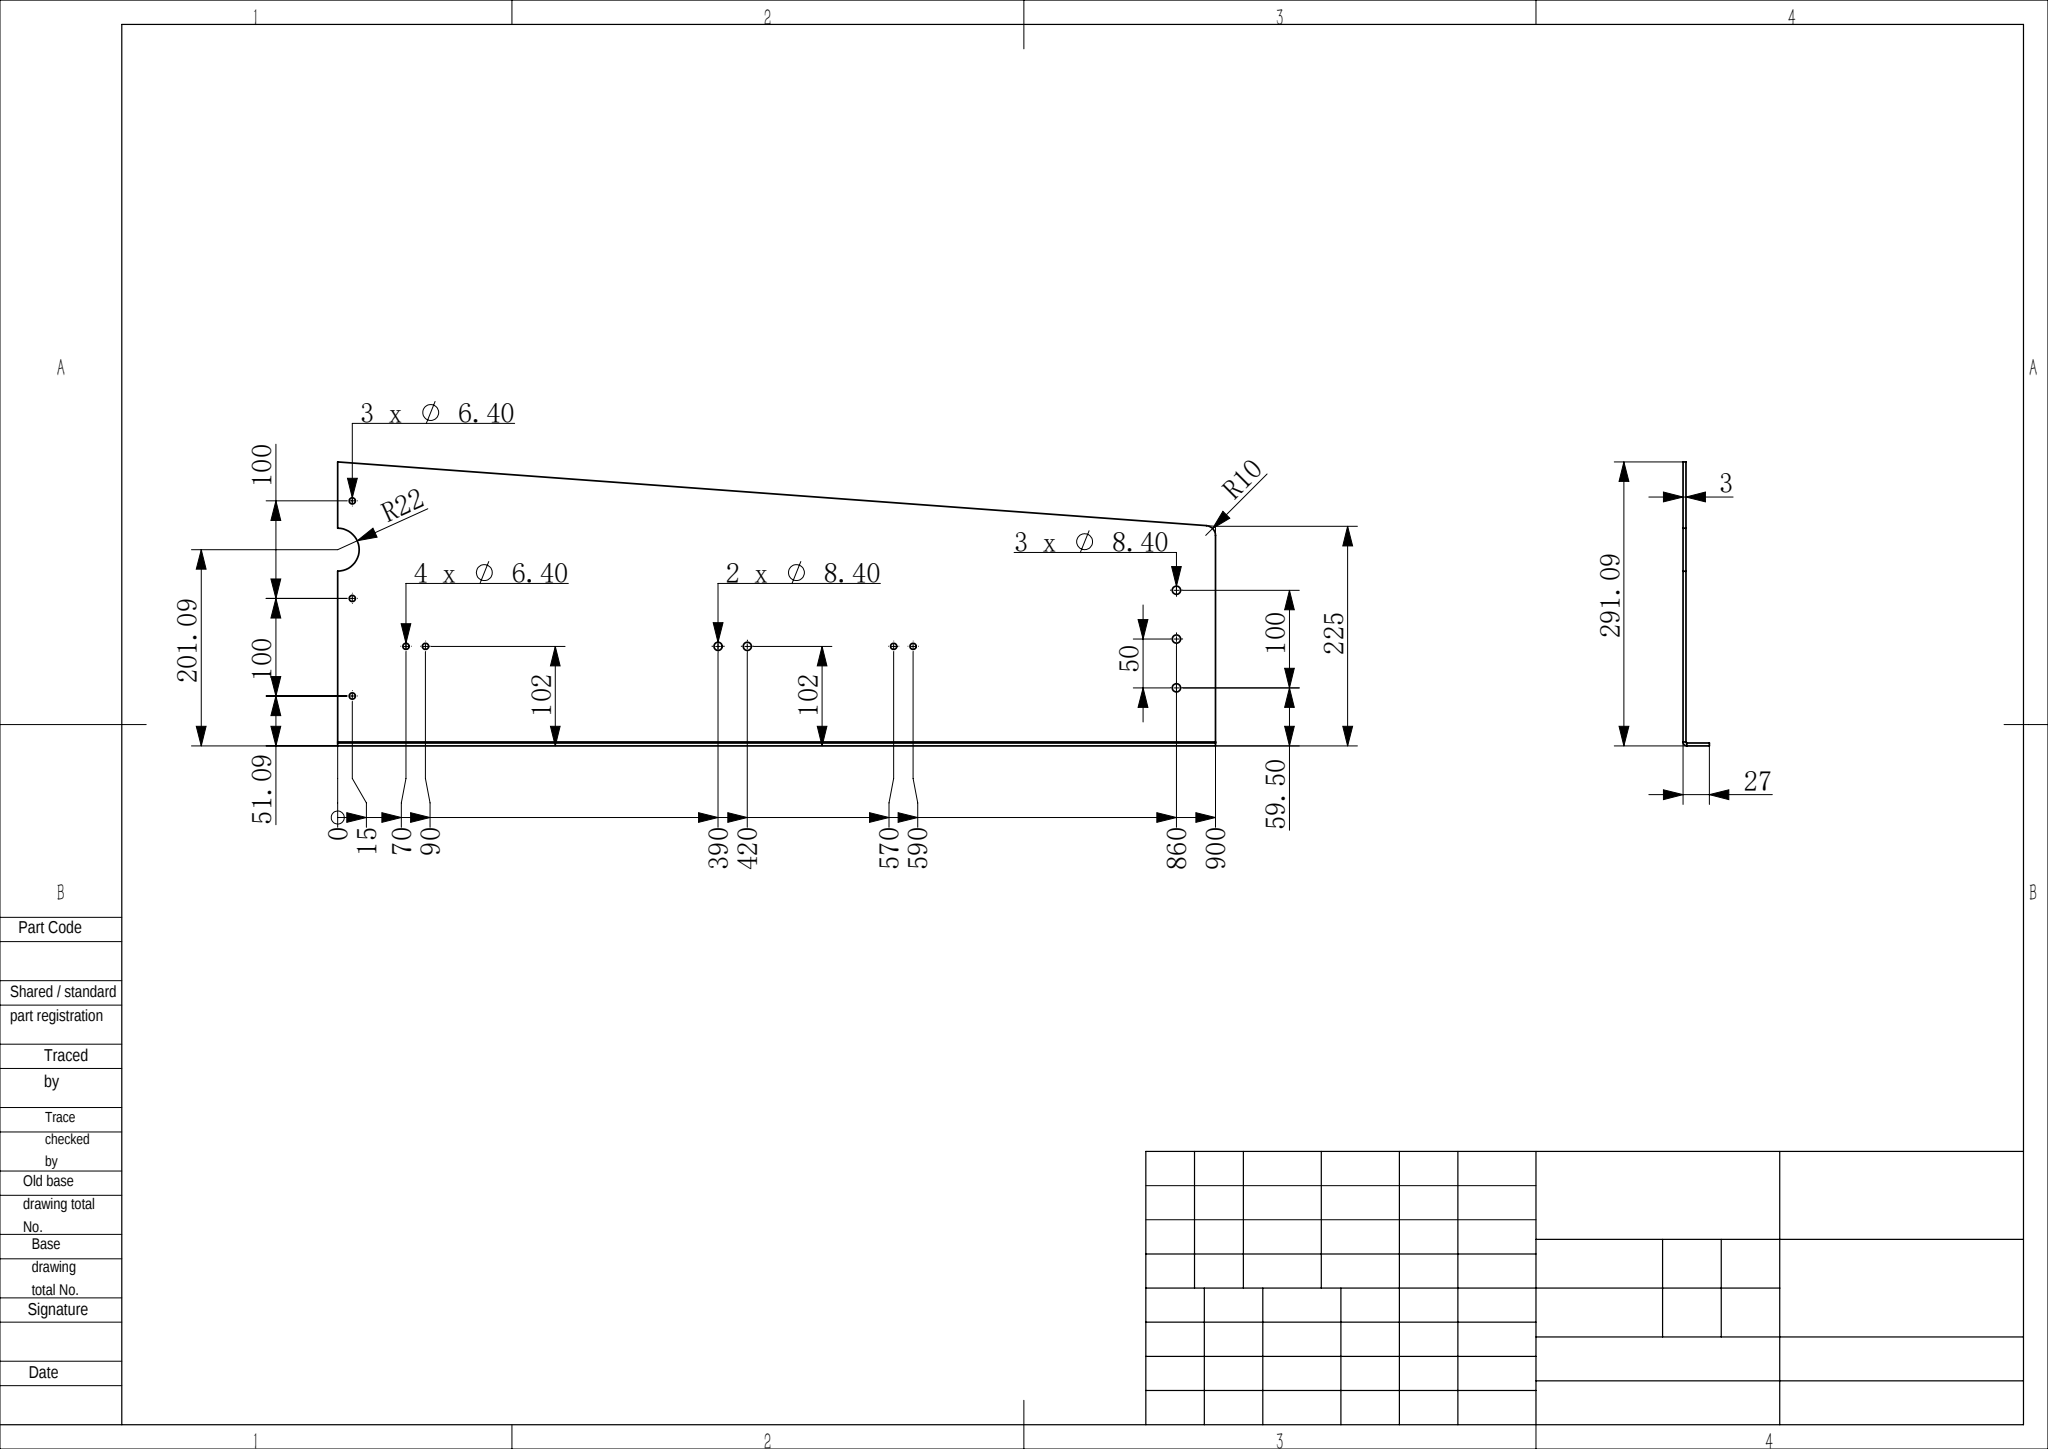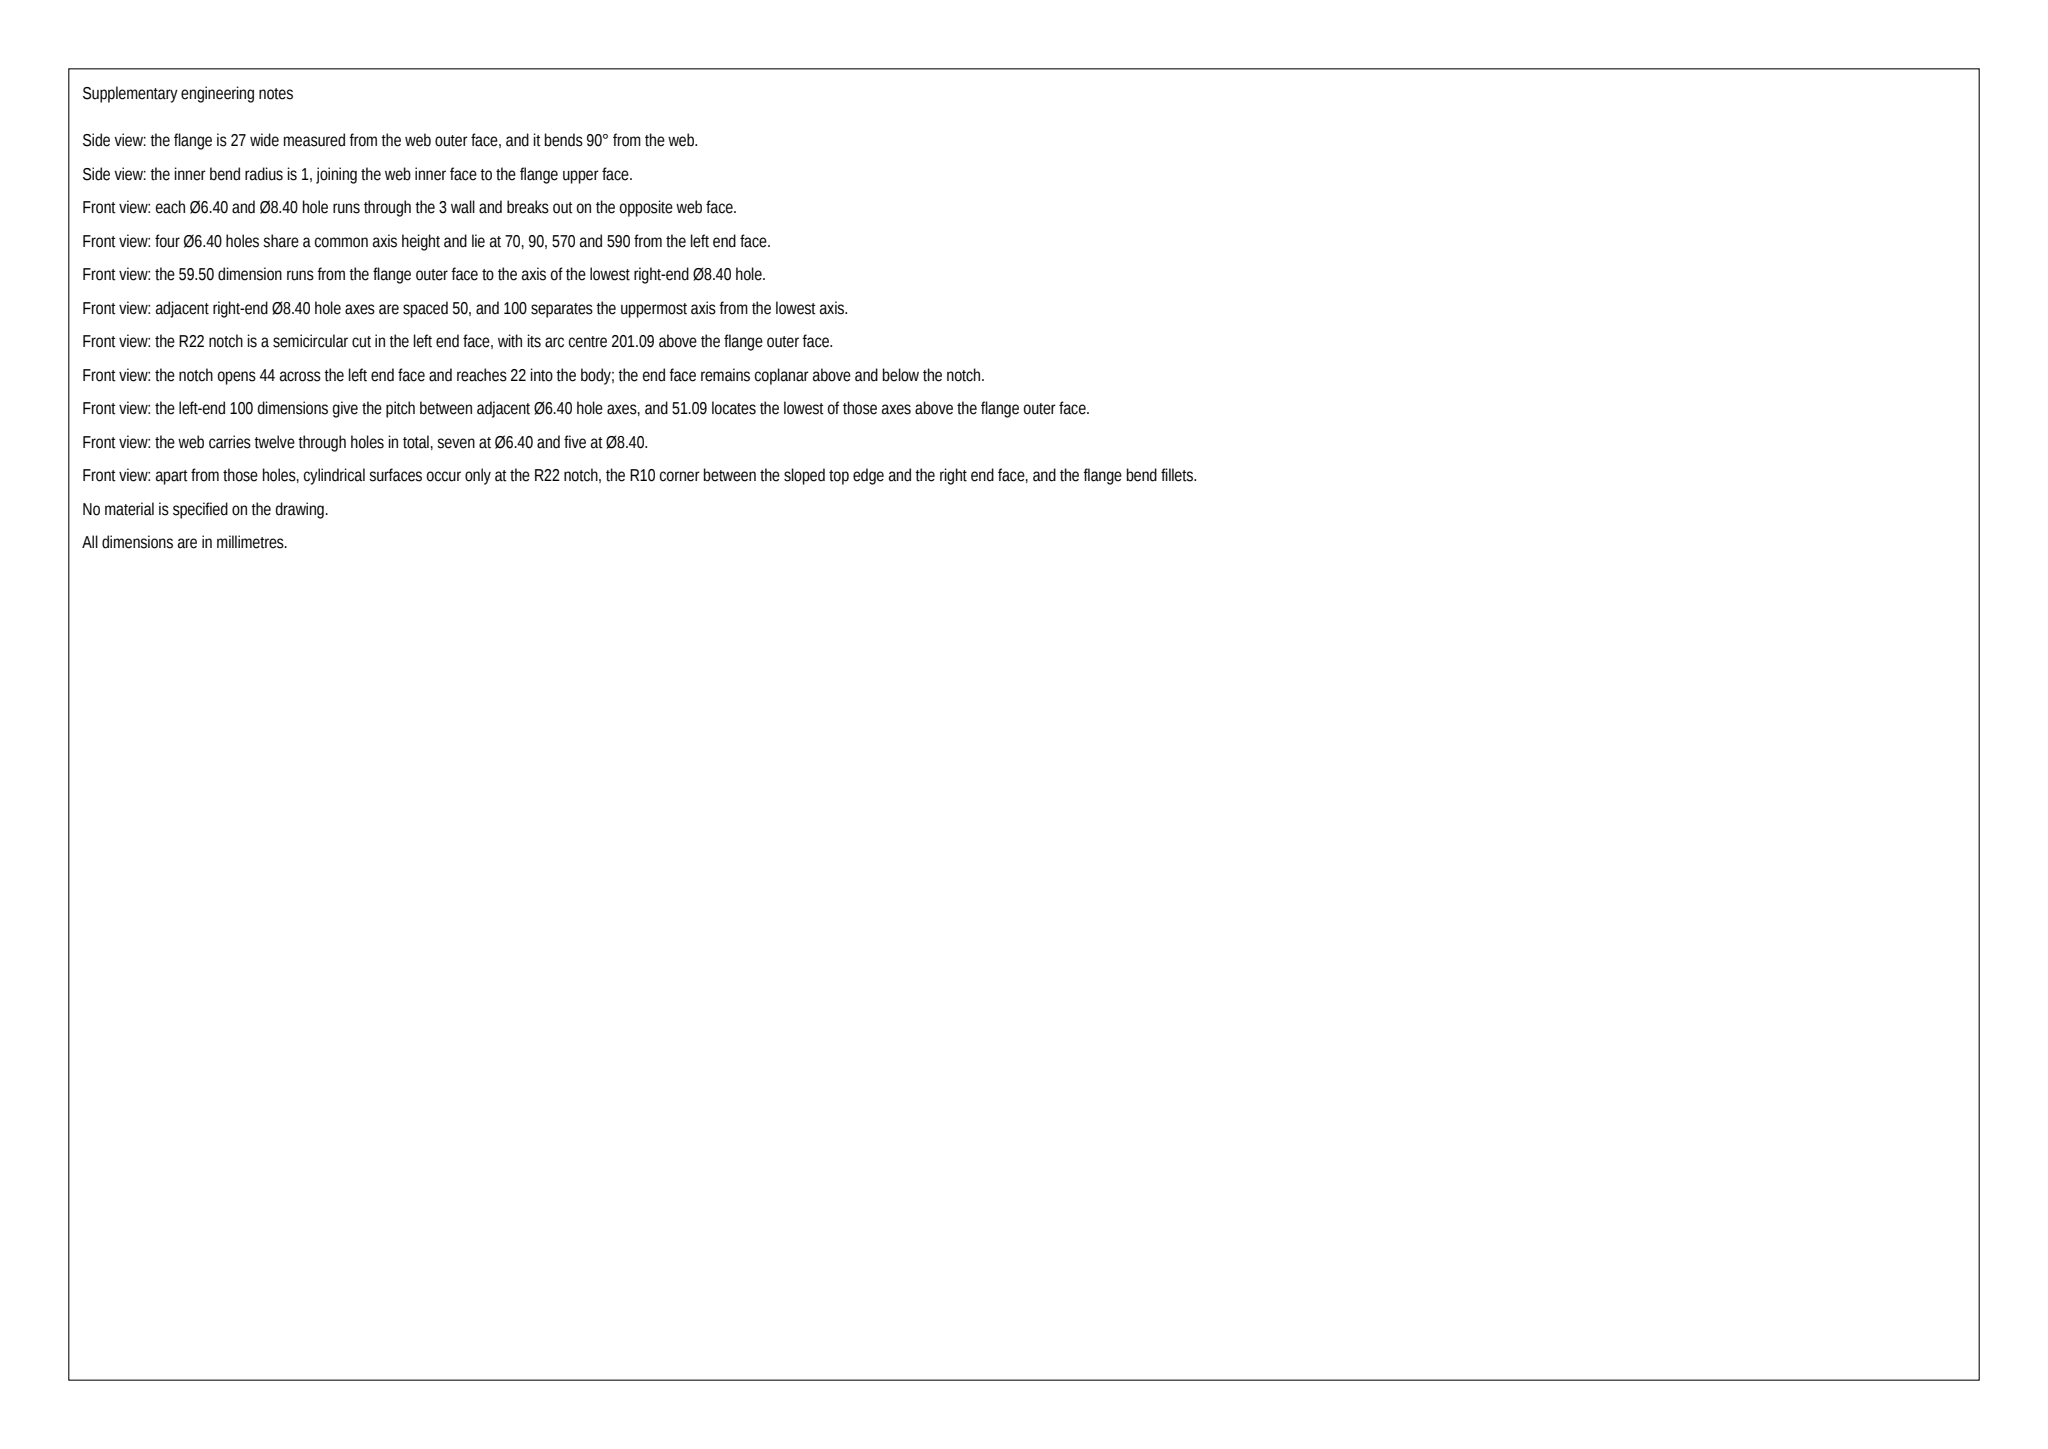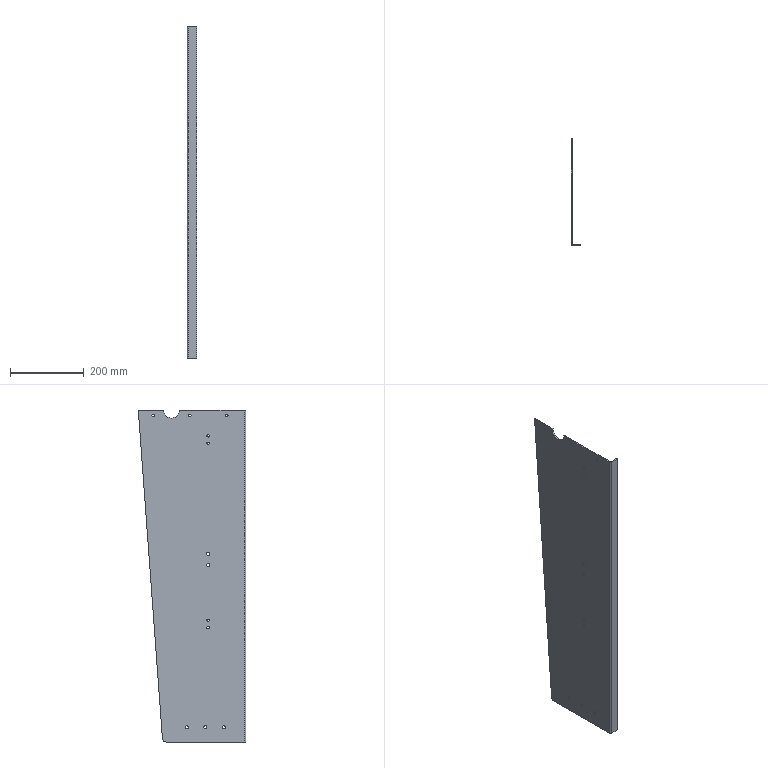Part | SolidWorks | mm | 1 solid | 42 faces | box 27 x 291.09 x 900 mm | volume 754785 mm3 | cylinder 29 | plane 13 | commonest cylinder face diameters 6.4 x14 8.4 x10 44 x2 8 x1 2 x1 20 x1